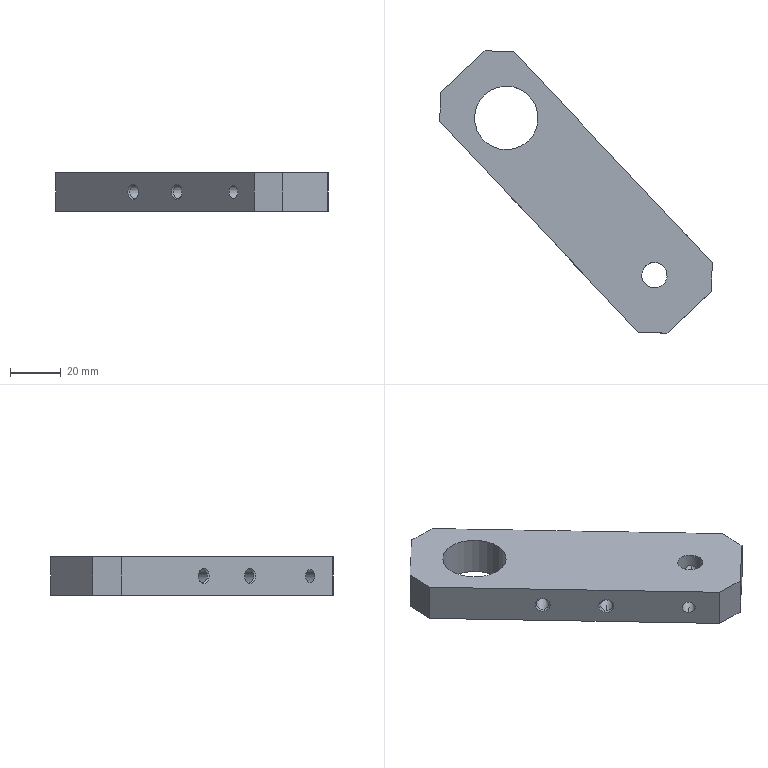Component | SolidWorks | RightSupportBlock-1 | 1 solid | 32 faces | box 107.26 x 111.11 x 15 mm | volume 66131 mm3 | cylinder 12 | cone 10 | plane 10 | commonest cylinder face diameters 5 x8 10 x2 25 x2
STEP:
#1=COLOUR_RGB('',0.7922,0.8196,0.9333);
#2=FILL_AREA_STYLE_COLOUR('',#1);
#3=FILL_AREA_STYLE('',(#2));
#4=SURFACE_STYLE_FILL_AREA(#3);
#5=SURFACE_SIDE_STYLE('',(#4));
#6=SURFACE_STYLE_USAGE(.BOTH.,#5);
#7=PRESENTATION_STYLE_ASSIGNMENT((#6));
#8=CARTESIAN_POINT('',(13.378,19.662,-9.461));
#9=VERTEX_POINT('',#8);
#10=CARTESIAN_POINT('',(13.378,19.662,-9.657));
#11=VERTEX_POINT('',#10);
#12=CARTESIAN_POINT('',(13.378,19.662,-9.559));
#13=DIRECTION('',(-0.7282,-0.6854,0.));
#14=DIRECTION('',(0.,0.,-1.));
#15=AXIS2_PLACEMENT_3D('',#12,#13,#14);
#16=CIRCLE('',#15,0.09843);
#17=EDGE_CURVE('',#9,#11,#16,.T.);
#18=ORIENTED_EDGE('',*,*,#17,.F.);
#19=CARTESIAN_POINT('',(13.363,19.648,-9.44));
#20=VERTEX_POINT('',#19);
#21=CARTESIAN_POINT('',(13.378,19.662,-9.461));
#22=DIRECTION('',(-0.5149,-0.4846,0.7071));
#23=VECTOR('',#22,39.37);
#24=LINE('',#21,#23);
#25=EDGE_CURVE('',#9,#20,#24,.T.);
#26=ORIENTED_EDGE('',*,*,#25,.T.);
#27=CARTESIAN_POINT('',(13.363,19.648,-9.678));
#28=VERTEX_POINT('',#27);
#29=CARTESIAN_POINT('',(13.363,19.648,-9.559));
#30=DIRECTION('',(0.7282,0.6854,-0.));
#31=DIRECTION('',(0.,0.,-1.));
#32=AXIS2_PLACEMENT_3D('',#29,#30,#31);
#33=CIRCLE('',#32,0.1191);
#34=EDGE_CURVE('',#28,#20,#33,.T.);
#35=ORIENTED_EDGE('',*,*,#34,.F.);
#36=CARTESIAN_POINT('',(13.378,19.662,-9.657));
#37=DIRECTION('',(-0.5149,-0.4846,-0.7071));
#38=VECTOR('',#37,39.37);
#39=LINE('',#36,#38);
#40=EDGE_CURVE('',#11,#28,#39,.T.);
#41=ORIENTED_EDGE('',*,*,#40,.F.);
#42=EDGE_LOOP('',(#18,#26,#35,#41));
#43=FACE_OUTER_BOUND('',#42,.T.);
#44=CARTESIAN_POINT('',(13.378,19.662,-9.559));
#45=DIRECTION('',(-0.7282,-0.6854,0.));
#46=DIRECTION('',(0.,0.,-1.));
#47=AXIS2_PLACEMENT_3D('',#44,#45,#46);
#48=CONICAL_SURFACE('',#47,0.09843,0.7854);
#49=ADVANCED_FACE('',(#43),#48,.F.);
#50=CARTESIAN_POINT('',(12.703,20.379,-9.461));
#51=VERTEX_POINT('',#50);
#52=CARTESIAN_POINT('',(12.703,20.379,-9.657));
#53=VERTEX_POINT('',#52);
#54=CARTESIAN_POINT('',(12.703,20.379,-9.559));
#55=DIRECTION('',(-0.7282,-0.6854,0.));
#56=DIRECTION('',(0.,0.,-1.));
#57=AXIS2_PLACEMENT_3D('',#54,#55,#56);
#58=CIRCLE('',#57,0.09843);
#59=EDGE_CURVE('',#51,#53,#58,.T.);
#60=ORIENTED_EDGE('',*,*,#59,.F.);
#61=CARTESIAN_POINT('',(12.688,20.365,-9.44));
#62=VERTEX_POINT('',#61);
#63=CARTESIAN_POINT('',(12.703,20.379,-9.461));
#64=DIRECTION('',(-0.5149,-0.4846,0.7071));
#65=VECTOR('',#64,39.37);
#66=LINE('',#63,#65);
#67=EDGE_CURVE('',#51,#62,#66,.T.);
#68=ORIENTED_EDGE('',*,*,#67,.T.);
#69=CARTESIAN_POINT('',(12.688,20.365,-9.678));
#70=VERTEX_POINT('',#69);
#71=CARTESIAN_POINT('',(12.688,20.365,-9.559));
#72=DIRECTION('',(0.7282,0.6854,-0.));
#73=DIRECTION('',(0.,0.,-1.));
#74=AXIS2_PLACEMENT_3D('',#71,#72,#73);
#75=CIRCLE('',#74,0.1191);
#76=EDGE_CURVE('',#70,#62,#75,.T.);
#77=ORIENTED_EDGE('',*,*,#76,.F.);
#78=CARTESIAN_POINT('',(12.703,20.379,-9.657));
#79=DIRECTION('',(-0.5149,-0.4846,-0.7071));
#80=VECTOR('',#79,39.37);
#81=LINE('',#78,#80);
#82=EDGE_CURVE('',#53,#70,#81,.T.);
#83=ORIENTED_EDGE('',*,*,#82,.F.);
#84=EDGE_LOOP('',(#60,#68,#77,#83));
#85=FACE_OUTER_BOUND('',#84,.T.);
#86=CARTESIAN_POINT('',(12.703,20.379,-9.559));
#87=DIRECTION('',(-0.7282,-0.6854,0.));
#88=DIRECTION('',(0.,0.,-1.));
#89=AXIS2_PLACEMENT_3D('',#86,#87,#88);
#90=CONICAL_SURFACE('',#89,0.09843,0.7854);
#91=ADVANCED_FACE('',(#85),#90,.F.);
#92=CARTESIAN_POINT('',(15.372,19.782,-9.657));
#93=VERTEX_POINT('',#92);
#94=CARTESIAN_POINT('',(15.372,19.782,-9.461));
#95=VERTEX_POINT('',#94);
#96=CARTESIAN_POINT('',(15.372,19.782,-9.559));
#97=DIRECTION('',(0.7282,0.6854,-0.));
#98=DIRECTION('',(0.,0.,1.));
#99=AXIS2_PLACEMENT_3D('',#96,#97,#98);
#100=CIRCLE('',#99,0.09843);
#101=EDGE_CURVE('',#93,#95,#100,.T.);
#102=ORIENTED_EDGE('',*,*,#101,.F.);
#103=CARTESIAN_POINT('',(15.387,19.796,-9.678));
#104=VERTEX_POINT('',#103);
#105=CARTESIAN_POINT('',(15.372,19.782,-9.657));
#106=DIRECTION('',(0.5149,0.4846,-0.7071));
#107=VECTOR('',#106,39.37);
#108=LINE('',#105,#107);
#109=EDGE_CURVE('',#93,#104,#108,.T.);
#110=ORIENTED_EDGE('',*,*,#109,.T.);
#111=CARTESIAN_POINT('',(15.387,19.796,-9.44));
#112=VERTEX_POINT('',#111);
#113=CARTESIAN_POINT('',(15.387,19.796,-9.559));
#114=DIRECTION('',(-0.7282,-0.6854,0.));
#115=DIRECTION('',(-0.6854,0.7282,0.));
#116=AXIS2_PLACEMENT_3D('',#113,#114,#115);
#117=CIRCLE('',#116,0.1191);
#118=EDGE_CURVE('',#112,#104,#117,.T.);
#119=ORIENTED_EDGE('',*,*,#118,.F.);
#120=CARTESIAN_POINT('',(15.372,19.782,-9.461));
#121=DIRECTION('',(0.5149,0.4846,0.7071));
#122=VECTOR('',#121,39.37);
#123=LINE('',#120,#122);
#124=EDGE_CURVE('',#95,#112,#123,.T.);
#125=ORIENTED_EDGE('',*,*,#124,.F.);
#126=EDGE_LOOP('',(#102,#110,#119,#125));
#127=FACE_OUTER_BOUND('',#126,.T.);
#128=CARTESIAN_POINT('',(15.372,19.782,-9.559));
#129=DIRECTION('',(0.7282,0.6854,-0.));
#130=DIRECTION('',(0.,0.,1.));
#131=AXIS2_PLACEMENT_3D('',#128,#129,#130);
#132=CONICAL_SURFACE('',#131,0.09843,0.7854);
#133=ADVANCED_FACE('',(#127),#132,.F.);
#134=CARTESIAN_POINT('',(13.262,20.905,-9.461));
#135=VERTEX_POINT('',#134);
#136=CARTESIAN_POINT('',(13.262,20.905,-9.657));
#137=VERTEX_POINT('',#136);
#138=CARTESIAN_POINT('',(13.262,20.905,-9.559));
#139=DIRECTION('',(-0.7282,-0.6854,0.));
#140=DIRECTION('',(0.,0.,-1.));
#141=AXIS2_PLACEMENT_3D('',#138,#139,#140);
#142=CIRCLE('',#141,0.09843);
#143=EDGE_CURVE('',#135,#137,#142,.T.);
#144=ORIENTED_EDGE('',*,*,#143,.F.);
#145=CARTESIAN_POINT('',(12.688,20.365,-9.461));
#146=DIRECTION('',(-0.7282,-0.6854,0.));
#147=VECTOR('',#146,39.37);
#148=LINE('',#145,#147);
#149=EDGE_CURVE('',#135,#51,#148,.T.);
#150=ORIENTED_EDGE('',*,*,#149,.T.);
#151=ORIENTED_EDGE('',*,*,#59,.T.);
#152=CARTESIAN_POINT('',(12.688,20.365,-9.657));
#153=DIRECTION('',(-0.7282,-0.6854,0.));
#154=VECTOR('',#153,39.37);
#155=LINE('',#152,#154);
#156=EDGE_CURVE('',#137,#53,#155,.T.);
#157=ORIENTED_EDGE('',*,*,#156,.F.);
#158=EDGE_LOOP('',(#144,#150,#151,#157));
#159=FACE_OUTER_BOUND('',#158,.T.);
#160=CARTESIAN_POINT('',(12.688,20.365,-9.559));
#161=DIRECTION('',(-0.7282,-0.6854,0.));
#162=DIRECTION('',(0.,0.,-1.));
#163=AXIS2_PLACEMENT_3D('',#160,#161,#162);
#164=CYLINDRICAL_SURFACE('',#163,0.09843);
#165=ADVANCED_FACE('',(#159),#164,.F.);
#166=CARTESIAN_POINT('',(13.305,20.945,-9.559));
#167=VERTEX_POINT('',#166);
#168=CARTESIAN_POINT('',(13.262,20.905,-9.657));
#169=DIRECTION('',(-0.375,-0.353,-0.8572));
#170=VECTOR('',#169,39.37);
#171=LINE('',#168,#170);
#172=EDGE_CURVE('',#167,#137,#171,.T.);
#173=ORIENTED_EDGE('',*,*,#172,.F.);
#174=CARTESIAN_POINT('',(13.262,20.905,-9.461));
#175=DIRECTION('',(-0.375,-0.353,0.8572));
#176=VECTOR('',#175,39.37);
#177=LINE('',#174,#176);
#178=EDGE_CURVE('',#167,#135,#177,.T.);
#179=ORIENTED_EDGE('',*,*,#178,.T.);
#180=ORIENTED_EDGE('',*,*,#143,.T.);
#181=EDGE_LOOP('',(#173,#179,#180));
#182=FACE_OUTER_BOUND('',#181,.T.);
#183=CARTESIAN_POINT('',(13.262,20.905,-9.559));
#184=DIRECTION('',(-0.7282,-0.6854,0.));
#185=DIRECTION('',(0.,0.,-1.));
#186=AXIS2_PLACEMENT_3D('',#183,#184,#185);
#187=CONICAL_SURFACE('',#186,0.09843,1.03);
#188=ADVANCED_FACE('',(#182),#187,.F.);
#189=CARTESIAN_POINT('',(13.936,20.188,-9.461));
#190=VERTEX_POINT('',#189);
#191=CARTESIAN_POINT('',(13.936,20.188,-9.657));
#192=VERTEX_POINT('',#191);
#193=CARTESIAN_POINT('',(13.936,20.188,-9.559));
#194=DIRECTION('',(-0.7282,-0.6854,0.));
#195=DIRECTION('',(0.,0.,-1.));
#196=AXIS2_PLACEMENT_3D('',#193,#194,#195);
#197=CIRCLE('',#196,0.09843);
#198=EDGE_CURVE('',#190,#192,#197,.T.);
#199=ORIENTED_EDGE('',*,*,#198,.F.);
#200=CARTESIAN_POINT('',(13.363,19.648,-9.461));
#201=DIRECTION('',(-0.7282,-0.6854,0.));
#202=VECTOR('',#201,39.37);
#203=LINE('',#200,#202);
#204=EDGE_CURVE('',#190,#9,#203,.T.);
#205=ORIENTED_EDGE('',*,*,#204,.T.);
#206=ORIENTED_EDGE('',*,*,#17,.T.);
#207=CARTESIAN_POINT('',(13.363,19.648,-9.657));
#208=DIRECTION('',(-0.7282,-0.6854,0.));
#209=VECTOR('',#208,39.37);
#210=LINE('',#207,#209);
#211=EDGE_CURVE('',#192,#11,#210,.T.);
#212=ORIENTED_EDGE('',*,*,#211,.F.);
#213=EDGE_LOOP('',(#199,#205,#206,#212));
#214=FACE_OUTER_BOUND('',#213,.T.);
#215=CARTESIAN_POINT('',(13.363,19.648,-9.559));
#216=DIRECTION('',(-0.7282,-0.6854,0.));
#217=DIRECTION('',(0.,0.,-1.));
#218=AXIS2_PLACEMENT_3D('',#215,#216,#217);
#219=CYLINDRICAL_SURFACE('',#218,0.09843);
#220=ADVANCED_FACE('',(#214),#219,.F.);
#221=CARTESIAN_POINT('',(13.979,20.228,-9.559));
#222=VERTEX_POINT('',#221);
#223=CARTESIAN_POINT('',(13.936,20.188,-9.657));
#224=DIRECTION('',(-0.375,-0.353,-0.8572));
#225=VECTOR('',#224,39.37);
#226=LINE('',#223,#225);
#227=EDGE_CURVE('',#222,#192,#226,.T.);
#228=ORIENTED_EDGE('',*,*,#227,.F.);
#229=CARTESIAN_POINT('',(13.936,20.188,-9.461));
#230=DIRECTION('',(-0.375,-0.353,0.8572));
#231=VECTOR('',#230,39.37);
#232=LINE('',#229,#231);
#233=EDGE_CURVE('',#222,#190,#232,.T.);
#234=ORIENTED_EDGE('',*,*,#233,.T.);
#235=ORIENTED_EDGE('',*,*,#198,.T.);
#236=EDGE_LOOP('',(#228,#234,#235));
#237=FACE_OUTER_BOUND('',#236,.T.);
#238=CARTESIAN_POINT('',(13.936,20.188,-9.559));
#239=DIRECTION('',(-0.7282,-0.6854,0.));
#240=DIRECTION('',(0.,0.,-1.));
#241=AXIS2_PLACEMENT_3D('',#238,#239,#240);
#242=CONICAL_SURFACE('',#241,0.09843,1.03);
#243=ADVANCED_FACE('',(#237),#242,.F.);
#244=CARTESIAN_POINT('',(14.24,18.716,-9.461));
#245=VERTEX_POINT('',#244);
#246=CARTESIAN_POINT('',(14.24,18.716,-9.657));
#247=VERTEX_POINT('',#246);
#248=CARTESIAN_POINT('',(14.24,18.716,-9.559));
#249=DIRECTION('',(-0.7282,-0.6854,0.));
#250=DIRECTION('',(0.,0.,-1.));
#251=AXIS2_PLACEMENT_3D('',#248,#249,#250);
#252=CIRCLE('',#251,0.09843);
#253=EDGE_CURVE('',#245,#247,#252,.T.);
#254=ORIENTED_EDGE('',*,*,#253,.T.);
#255=CARTESIAN_POINT('',(14.67,19.121,-9.657));
#256=VERTEX_POINT('',#255);
#257=CARTESIAN_POINT('',(15.387,19.796,-9.657));
#258=DIRECTION('',(0.7282,0.6854,-0.));
#259=VECTOR('',#258,39.37);
#260=LINE('',#257,#259);
#261=EDGE_CURVE('',#247,#256,#260,.T.);
#262=ORIENTED_EDGE('',*,*,#261,.T.);
#263=CARTESIAN_POINT('',(14.67,19.121,-9.461));
#264=VERTEX_POINT('',#263);
#265=CARTESIAN_POINT('',(14.67,19.121,-9.461));
#266=CARTESIAN_POINT('',(14.665,19.126,-9.461));
#267=CARTESIAN_POINT('',(14.661,19.131,-9.461));
#268=CARTESIAN_POINT('',(14.653,19.141,-9.464));
#269=CARTESIAN_POINT('',(14.65,19.146,-9.466));
#270=CARTESIAN_POINT('',(14.64,19.162,-9.473));
#271=CARTESIAN_POINT('',(14.635,19.172,-9.481));
#272=CARTESIAN_POINT('',(14.63,19.185,-9.494));
#273=CARTESIAN_POINT('',(14.628,19.189,-9.499));
#274=CARTESIAN_POINT('',(14.626,19.197,-9.51));
#275=CARTESIAN_POINT('',(14.625,19.2,-9.515));
#276=CARTESIAN_POINT('',(14.623,19.205,-9.527));
#277=CARTESIAN_POINT('',(14.623,19.207,-9.533));
#278=CARTESIAN_POINT('',(14.622,19.21,-9.546));
#279=CARTESIAN_POINT('',(14.622,19.211,-9.552));
#280=CARTESIAN_POINT('',(14.622,19.211,-9.566));
#281=CARTESIAN_POINT('',(14.622,19.21,-9.572));
#282=CARTESIAN_POINT('',(14.623,19.207,-9.585));
#283=CARTESIAN_POINT('',(14.623,19.205,-9.591));
#284=CARTESIAN_POINT('',(14.625,19.2,-9.603));
#285=CARTESIAN_POINT('',(14.626,19.197,-9.609));
#286=CARTESIAN_POINT('',(14.628,19.189,-9.619));
#287=CARTESIAN_POINT('',(14.63,19.185,-9.624));
#288=CARTESIAN_POINT('',(14.635,19.172,-9.638));
#289=CARTESIAN_POINT('',(14.64,19.162,-9.645));
#290=CARTESIAN_POINT('',(14.65,19.146,-9.652));
#291=CARTESIAN_POINT('',(14.653,19.141,-9.654));
#292=CARTESIAN_POINT('',(14.661,19.131,-9.657));
#293=CARTESIAN_POINT('',(14.665,19.126,-9.657));
#294=CARTESIAN_POINT('',(14.67,19.121,-9.657));
#295=B_SPLINE_CURVE_WITH_KNOTS('',3,(#265,#266,#267,#268,#269,#270,#271,#272,#273,#274,#275,#276,#277,#278,#279,#280,#281,#282,#283,#284,#285,#286,#287,#288,#289,#290,#291,#292,#293,#294),.UNSPECIFIED.,.F.,.F.,(4,2,2,2,2,2,2,2,2,2,2,2,2,2,4),(0.,0.000497,0.0009941,0.001988,0.002485,0.002982,0.003479,0.003976,0.004473,0.00497,0.005467,0.005964,0.006958,0.007455,0.007952),.UNSPECIFIED.);
#296=EDGE_CURVE('',#264,#256,#295,.T.);
#297=ORIENTED_EDGE('',*,*,#296,.F.);
#298=CARTESIAN_POINT('',(15.387,19.796,-9.461));
#299=DIRECTION('',(0.7282,0.6854,-0.));
#300=VECTOR('',#299,39.37);
#301=LINE('',#298,#300);
#302=EDGE_CURVE('',#245,#264,#301,.T.);
#303=ORIENTED_EDGE('',*,*,#302,.F.);
#304=EDGE_LOOP('',(#254,#262,#297,#303));
#305=FACE_OUTER_BOUND('',#304,.T.);
#306=CARTESIAN_POINT('',(15.387,19.796,-9.559));
#307=DIRECTION('',(0.7282,0.6854,-0.));
#308=DIRECTION('',(0.,0.,1.));
#309=AXIS2_PLACEMENT_3D('',#306,#307,#308);
#310=CYLINDRICAL_SURFACE('',#309,0.09843);
#311=ADVANCED_FACE('',(#305),#310,.F.);
#312=CARTESIAN_POINT('',(14.957,19.391,-9.657));
#313=VERTEX_POINT('',#312);
#314=CARTESIAN_POINT('',(14.957,19.391,-9.461));
#315=VERTEX_POINT('',#314);
#316=CARTESIAN_POINT('',(14.957,19.391,-9.657));
#317=CARTESIAN_POINT('',(14.952,19.396,-9.657));
#318=CARTESIAN_POINT('',(14.947,19.4,-9.657));
#319=CARTESIAN_POINT('',(14.938,19.409,-9.654));
#320=CARTESIAN_POINT('',(14.933,19.413,-9.652));
#321=CARTESIAN_POINT('',(14.923,19.42,-9.647));
#322=CARTESIAN_POINT('',(14.918,19.423,-9.644));
#323=CARTESIAN_POINT('',(14.909,19.428,-9.637));
#324=CARTESIAN_POINT('',(14.904,19.431,-9.633));
#325=CARTESIAN_POINT('',(14.895,19.435,-9.624));
#326=CARTESIAN_POINT('',(14.891,19.437,-9.619));
#327=CARTESIAN_POINT('',(14.884,19.44,-9.609));
#328=CARTESIAN_POINT('',(14.881,19.441,-9.603));
#329=CARTESIAN_POINT('',(14.876,19.443,-9.591));
#330=CARTESIAN_POINT('',(14.874,19.443,-9.585));
#331=CARTESIAN_POINT('',(14.871,19.444,-9.572));
#332=CARTESIAN_POINT('',(14.87,19.445,-9.566));
#333=CARTESIAN_POINT('',(14.87,19.445,-9.553));
#334=CARTESIAN_POINT('',(14.871,19.444,-9.546));
#335=CARTESIAN_POINT('',(14.874,19.444,-9.533));
#336=CARTESIAN_POINT('',(14.876,19.443,-9.527));
#337=CARTESIAN_POINT('',(14.884,19.44,-9.509));
#338=CARTESIAN_POINT('',(14.891,19.437,-9.499));
#339=CARTESIAN_POINT('',(14.904,19.431,-9.485));
#340=CARTESIAN_POINT('',(14.908,19.428,-9.481));
#341=CARTESIAN_POINT('',(14.918,19.423,-9.474));
#342=CARTESIAN_POINT('',(14.923,19.42,-9.471));
#343=CARTESIAN_POINT('',(14.933,19.413,-9.466));
#344=CARTESIAN_POINT('',(14.938,19.409,-9.464));
#345=CARTESIAN_POINT('',(14.947,19.4,-9.461));
#346=CARTESIAN_POINT('',(14.952,19.396,-9.461));
#347=CARTESIAN_POINT('',(14.957,19.391,-9.461));
#348=B_SPLINE_CURVE_WITH_KNOTS('',3,(#316,#317,#318,#319,#320,#321,#322,#323,#324,#325,#326,#327,#328,#329,#330,#331,#332,#333,#334,#335,#336,#337,#338,#339,#340,#341,#342,#343,#344,#345,#346,#347),.UNSPECIFIED.,.F.,.F.,(4,2,2,2,2,2,2,2,2,2,2,2,2,2,2,4),(0.007952,0.008449,0.008945,0.009441,0.009937,0.01043,0.01093,0.01143,0.01192,0.01242,0.01291,0.01391,0.0144,0.0149,0.01539,0.01589),.UNSPECIFIED.);
#349=EDGE_CURVE('',#313,#315,#348,.T.);
#350=ORIENTED_EDGE('',*,*,#349,.F.);
#351=CARTESIAN_POINT('',(15.387,19.796,-9.657));
#352=DIRECTION('',(0.7282,0.6854,-0.));
#353=VECTOR('',#352,39.37);
#354=LINE('',#351,#353);
#355=EDGE_CURVE('',#313,#93,#354,.T.);
#356=ORIENTED_EDGE('',*,*,#355,.T.);
#357=ORIENTED_EDGE('',*,*,#101,.T.);
#358=CARTESIAN_POINT('',(15.387,19.796,-9.461));
#359=DIRECTION('',(0.7282,0.6854,-0.));
#360=VECTOR('',#359,39.37);
#361=LINE('',#358,#360);
#362=EDGE_CURVE('',#315,#95,#361,.T.);
#363=ORIENTED_EDGE('',*,*,#362,.F.);
#364=EDGE_LOOP('',(#350,#356,#357,#363));
#365=FACE_OUTER_BOUND('',#364,.T.);
#366=CARTESIAN_POINT('',(15.387,19.796,-9.559));
#367=DIRECTION('',(0.7282,0.6854,-0.));
#368=DIRECTION('',(0.,0.,1.));
#369=AXIS2_PLACEMENT_3D('',#366,#367,#368);
#370=CYLINDRICAL_SURFACE('',#369,0.09843);
#371=ADVANCED_FACE('',(#365),#370,.F.);
#372=ORIENTED_EDGE('',*,*,#296,.T.);
#373=CARTESIAN_POINT('',(14.67,19.121,-9.657));
#374=CARTESIAN_POINT('',(14.674,19.116,-9.657));
#375=CARTESIAN_POINT('',(14.679,19.112,-9.657));
#376=CARTESIAN_POINT('',(14.689,19.103,-9.654));
#377=CARTESIAN_POINT('',(14.694,19.1,-9.652));
#378=CARTESIAN_POINT('',(14.704,19.092,-9.647));
#379=CARTESIAN_POINT('',(14.709,19.089,-9.644));
#380=CARTESIAN_POINT('',(14.718,19.084,-9.637));
#381=CARTESIAN_POINT('',(14.723,19.081,-9.633));
#382=CARTESIAN_POINT('',(14.731,19.077,-9.624));
#383=CARTESIAN_POINT('',(14.735,19.075,-9.619));
#384=CARTESIAN_POINT('',(14.742,19.072,-9.609));
#385=CARTESIAN_POINT('',(14.746,19.071,-9.603));
#386=CARTESIAN_POINT('',(14.751,19.069,-9.591));
#387=CARTESIAN_POINT('',(14.753,19.069,-9.585));
#388=CARTESIAN_POINT('',(14.756,19.068,-9.572));
#389=CARTESIAN_POINT('',(14.757,19.068,-9.566));
#390=CARTESIAN_POINT('',(14.757,19.068,-9.553));
#391=CARTESIAN_POINT('',(14.756,19.068,-9.546));
#392=CARTESIAN_POINT('',(14.753,19.069,-9.533));
#393=CARTESIAN_POINT('',(14.751,19.069,-9.527));
#394=CARTESIAN_POINT('',(14.743,19.072,-9.509));
#395=CARTESIAN_POINT('',(14.736,19.075,-9.499));
#396=CARTESIAN_POINT('',(14.723,19.081,-9.485));
#397=CARTESIAN_POINT('',(14.718,19.084,-9.481));
#398=CARTESIAN_POINT('',(14.709,19.089,-9.474));
#399=CARTESIAN_POINT('',(14.704,19.092,-9.471));
#400=CARTESIAN_POINT('',(14.694,19.099,-9.466));
#401=CARTESIAN_POINT('',(14.689,19.103,-9.464));
#402=CARTESIAN_POINT('',(14.679,19.112,-9.461));
#403=CARTESIAN_POINT('',(14.674,19.116,-9.461));
#404=CARTESIAN_POINT('',(14.67,19.121,-9.461));
#405=B_SPLINE_CURVE_WITH_KNOTS('',3,(#373,#374,#375,#376,#377,#378,#379,#380,#381,#382,#383,#384,#385,#386,#387,#388,#389,#390,#391,#392,#393,#394,#395,#396,#397,#398,#399,#400,#401,#402,#403,#404),.UNSPECIFIED.,.F.,.F.,(4,2,2,2,2,2,2,2,2,2,2,2,2,2,2,4),(0.007952,0.008449,0.008945,0.009441,0.009937,0.01043,0.01093,0.01143,0.01192,0.01242,0.01291,0.01391,0.0144,0.0149,0.01539,0.01589),.UNSPECIFIED.);
#406=EDGE_CURVE('',#256,#264,#405,.T.);
#407=ORIENTED_EDGE('',*,*,#406,.T.);
#408=EDGE_LOOP('',(#372,#407));
#409=FACE_BOUND('',#408,.T.);
#410=CARTESIAN_POINT('',(14.678,19.399,-9.854));
#411=VERTEX_POINT('',#410);
#412=CARTESIAN_POINT('',(14.948,19.113,-9.854));
#413=VERTEX_POINT('',#412);
#414=CARTESIAN_POINT('',(14.813,19.256,-9.854));
#415=DIRECTION('',(-0.,0.,1.));
#416=DIRECTION('',(0.6854,-0.7282,0.));
#417=AXIS2_PLACEMENT_3D('',#414,#415,#416);
#418=CIRCLE('',#417,0.1969);
#419=EDGE_CURVE('',#411,#413,#418,.T.);
#420=ORIENTED_EDGE('',*,*,#419,.F.);
#421=CARTESIAN_POINT('',(14.678,19.399,-9.264));
#422=VERTEX_POINT('',#421);
#423=CARTESIAN_POINT('',(14.678,19.399,-9.264));
#424=DIRECTION('',(-0.,0.,1.));
#425=VECTOR('',#424,39.37);
#426=LINE('',#423,#425);
#427=EDGE_CURVE('',#411,#422,#426,.T.);
#428=ORIENTED_EDGE('',*,*,#427,.T.);
#429=CARTESIAN_POINT('',(14.948,19.113,-9.264));
#430=VERTEX_POINT('',#429);
#431=CARTESIAN_POINT('',(14.813,19.256,-9.264));
#432=DIRECTION('',(-0.,0.,1.));
#433=DIRECTION('',(0.6854,-0.7282,0.));
#434=AXIS2_PLACEMENT_3D('',#431,#432,#433);
#435=CIRCLE('',#434,0.1969);
#436=EDGE_CURVE('',#422,#430,#435,.T.);
#437=ORIENTED_EDGE('',*,*,#436,.T.);
#438=CARTESIAN_POINT('',(14.948,19.113,-9.264));
#439=DIRECTION('',(-0.,0.,1.));
#440=VECTOR('',#439,39.37);
#441=LINE('',#438,#440);
#442=EDGE_CURVE('',#413,#430,#441,.T.);
#443=ORIENTED_EDGE('',*,*,#442,.F.);
#444=EDGE_LOOP('',(#420,#428,#437,#443));
#445=FACE_OUTER_BOUND('',#444,.T.);
#446=CARTESIAN_POINT('',(14.813,19.256,-9.264));
#447=DIRECTION('',(-0.,0.,1.));
#448=DIRECTION('',(0.6854,-0.7282,0.));
#449=AXIS2_PLACEMENT_3D('',#446,#447,#448);
#450=CYLINDRICAL_SURFACE('',#449,0.1969);
#451=ADVANCED_FACE('',(#409,#445),#450,.F.);
#452=CARTESIAN_POINT('',(12.182,22.051,-9.854));
#453=VERTEX_POINT('',#452);
#454=CARTESIAN_POINT('',(12.857,21.335,-9.854));
#455=VERTEX_POINT('',#454);
#456=CARTESIAN_POINT('',(12.52,21.693,-9.854));
#457=DIRECTION('',(-0.,0.,1.));
#458=DIRECTION('',(0.6854,-0.7282,0.));
#459=AXIS2_PLACEMENT_3D('',#456,#457,#458);
#460=CIRCLE('',#459,0.4921);
#461=EDGE_CURVE('',#453,#455,#460,.T.);
#462=ORIENTED_EDGE('',*,*,#461,.F.);
#463=CARTESIAN_POINT('',(12.182,22.051,-9.264));
#464=VERTEX_POINT('',#463);
#465=CARTESIAN_POINT('',(12.182,22.051,-9.264));
#466=DIRECTION('',(-0.,0.,1.));
#467=VECTOR('',#466,39.37);
#468=LINE('',#465,#467);
#469=EDGE_CURVE('',#453,#464,#468,.T.);
#470=ORIENTED_EDGE('',*,*,#469,.T.);
#471=CARTESIAN_POINT('',(12.857,21.335,-9.264));
#472=VERTEX_POINT('',#471);
#473=CARTESIAN_POINT('',(12.52,21.693,-9.264));
#474=DIRECTION('',(-0.,0.,1.));
#475=DIRECTION('',(0.6854,-0.7282,0.));
#476=AXIS2_PLACEMENT_3D('',#473,#474,#475);
#477=CIRCLE('',#476,0.4921);
#478=EDGE_CURVE('',#464,#472,#477,.T.);
#479=ORIENTED_EDGE('',*,*,#478,.T.);
#480=CARTESIAN_POINT('',(12.857,21.335,-9.264));
#481=DIRECTION('',(-0.,0.,1.));
#482=VECTOR('',#481,39.37);
#483=LINE('',#480,#482);
#484=EDGE_CURVE('',#455,#472,#483,.T.);
#485=ORIENTED_EDGE('',*,*,#484,.F.);
#486=EDGE_LOOP('',(#462,#470,#479,#485));
#487=FACE_OUTER_BOUND('',#486,.T.);
#488=CARTESIAN_POINT('',(12.52,21.693,-9.264));
#489=DIRECTION('',(-0.,0.,1.));
#490=DIRECTION('',(0.6854,-0.7282,0.));
#491=AXIS2_PLACEMENT_3D('',#488,#489,#490);
#492=CYLINDRICAL_SURFACE('',#491,0.4921);
#493=ADVANCED_FACE('',(#487),#492,.F.);
#494=CARTESIAN_POINT('',(15.697,19.007,-9.264));
#495=VERTEX_POINT('',#494);
#496=CARTESIAN_POINT('',(15.009,18.359,-9.264));
#497=VERTEX_POINT('',#496);
#498=CARTESIAN_POINT('',(15.926,19.222,-9.264));
#499=DIRECTION('',(-0.7282,-0.6854,0.));
#500=VECTOR('',#499,39.37);
#501=LINE('',#498,#500);
#502=EDGE_CURVE('',#495,#497,#501,.T.);
#503=ORIENTED_EDGE('',*,*,#502,.T.);
#504=CARTESIAN_POINT('',(15.009,18.359,-9.854));
#505=VERTEX_POINT('',#504);
#506=CARTESIAN_POINT('',(15.009,18.359,-9.264));
#507=DIRECTION('',(0.,-0.,-1.));
#508=VECTOR('',#507,39.37);
#509=LINE('',#506,#508);
#510=EDGE_CURVE('',#497,#505,#509,.T.);
#511=ORIENTED_EDGE('',*,*,#510,.T.);
#512=CARTESIAN_POINT('',(15.697,19.007,-9.854));
#513=VERTEX_POINT('',#512);
#514=CARTESIAN_POINT('',(15.926,19.222,-9.854));
#515=DIRECTION('',(-0.7282,-0.6854,0.));
#516=VECTOR('',#515,39.37);
#517=LINE('',#514,#516);
#518=EDGE_CURVE('',#513,#505,#517,.T.);
#519=ORIENTED_EDGE('',*,*,#518,.F.);
#520=CARTESIAN_POINT('',(15.697,19.007,-9.264));
#521=DIRECTION('',(-0.,0.,1.));
#522=VECTOR('',#521,39.37);
#523=LINE('',#520,#522);
#524=EDGE_CURVE('',#513,#495,#523,.T.);
#525=ORIENTED_EDGE('',*,*,#524,.T.);
#526=EDGE_LOOP('',(#503,#511,#519,#525));
#527=FACE_OUTER_BOUND('',#526,.T.);
#528=CARTESIAN_POINT('',(15.926,19.222,-9.264));
#529=DIRECTION('',(0.6854,-0.7282,0.));
#530=DIRECTION('',(0.,-0.,-1.));
#531=AXIS2_PLACEMENT_3D('',#528,#529,#530);
#532=PLANE('',#531);
#533=ADVANCED_FACE('',(#527),#532,.T.);
#534=ORIENTED_EDGE('',*,*,#118,.T.);
#535=CARTESIAN_POINT('',(15.387,19.796,-9.559));
#536=DIRECTION('',(-0.7282,-0.6854,0.));
#537=DIRECTION('',(-0.6854,0.7282,0.));
#538=AXIS2_PLACEMENT_3D('',#535,#536,#537);
#539=CIRCLE('',#538,0.1191);
#540=EDGE_CURVE('',#104,#112,#539,.T.);
#541=ORIENTED_EDGE('',*,*,#540,.T.);
#542=EDGE_LOOP('',(#534,#541));
#543=FACE_BOUND('',#542,.T.);
#544=CARTESIAN_POINT('',(12.634,22.72,-9.854));
#545=VERTEX_POINT('',#544);
#546=CARTESIAN_POINT('',(15.71,19.452,-9.854));
#547=VERTEX_POINT('',#546);
#548=CARTESIAN_POINT('',(12.418,22.949,-9.854));
#549=DIRECTION('',(0.6854,-0.7282,0.));
#550=VECTOR('',#549,39.37);
#551=LINE('',#548,#550);
#552=EDGE_CURVE('',#545,#547,#551,.T.);
#553=ORIENTED_EDGE('',*,*,#552,.F.);
#554=CARTESIAN_POINT('',(12.634,22.72,-9.264));
#555=VERTEX_POINT('',#554);
#556=CARTESIAN_POINT('',(12.634,22.72,-9.264));
#557=DIRECTION('',(-0.,0.,1.));
#558=VECTOR('',#557,39.37);
#559=LINE('',#556,#558);
#560=EDGE_CURVE('',#545,#555,#559,.T.);
#561=ORIENTED_EDGE('',*,*,#560,.T.);
#562=CARTESIAN_POINT('',(15.71,19.452,-9.264));
#563=VERTEX_POINT('',#562);
#564=CARTESIAN_POINT('',(12.418,22.949,-9.264));
#565=DIRECTION('',(0.6854,-0.7282,0.));
#566=VECTOR('',#565,39.37);
#567=LINE('',#564,#566);
#568=EDGE_CURVE('',#555,#563,#567,.T.);
#569=ORIENTED_EDGE('',*,*,#568,.T.);
#570=CARTESIAN_POINT('',(15.71,19.452,-9.264));
#571=DIRECTION('',(0.,-0.,-1.));
#572=VECTOR('',#571,39.37);
#573=LINE('',#570,#572);
#574=EDGE_CURVE('',#563,#547,#573,.T.);
#575=ORIENTED_EDGE('',*,*,#574,.T.);
#576=EDGE_LOOP('',(#553,#561,#569,#575));
#577=FACE_OUTER_BOUND('',#576,.T.);
#578=CARTESIAN_POINT('',(12.418,22.949,-9.264));
#579=DIRECTION('',(0.7282,0.6854,-0.));
#580=DIRECTION('',(-0.6854,0.7282,-0.));
#581=AXIS2_PLACEMENT_3D('',#578,#579,#580);
#582=PLANE('',#581);
#583=ADVANCED_FACE('',(#543,#577),#582,.T.);
#584=CARTESIAN_POINT('',(11.501,22.086,-9.854));
#585=VERTEX_POINT('',#584);
#586=CARTESIAN_POINT('',(12.189,22.733,-9.854));
#587=VERTEX_POINT('',#586);
#588=CARTESIAN_POINT('',(11.272,21.87,-9.854));
#589=DIRECTION('',(0.7282,0.6854,-0.));
#590=VECTOR('',#589,39.37);
#591=LINE('',#588,#590);
#592=EDGE_CURVE('',#585,#587,#591,.T.);
#593=ORIENTED_EDGE('',*,*,#592,.F.);
#594=CARTESIAN_POINT('',(11.501,22.086,-9.264));
#595=VERTEX_POINT('',#594);
#596=CARTESIAN_POINT('',(11.501,22.086,-9.264));
#597=DIRECTION('',(-0.,0.,1.));
#598=VECTOR('',#597,39.37);
#599=LINE('',#596,#598);
#600=EDGE_CURVE('',#585,#595,#599,.T.);
#601=ORIENTED_EDGE('',*,*,#600,.T.);
#602=CARTESIAN_POINT('',(12.189,22.733,-9.264));
#603=VERTEX_POINT('',#602);
#604=CARTESIAN_POINT('',(11.272,21.87,-9.264));
#605=DIRECTION('',(0.7282,0.6854,-0.));
#606=VECTOR('',#605,39.37);
#607=LINE('',#604,#606);
#608=EDGE_CURVE('',#595,#603,#607,.T.);
#609=ORIENTED_EDGE('',*,*,#608,.T.);
#610=CARTESIAN_POINT('',(12.189,22.733,-9.264));
#611=DIRECTION('',(0.,-0.,-1.));
#612=VECTOR('',#611,39.37);
#613=LINE('',#610,#612);
#614=EDGE_CURVE('',#603,#587,#613,.T.);
#615=ORIENTED_EDGE('',*,*,#614,.T.);
#616=EDGE_LOOP('',(#593,#601,#609,#615));
#617=FACE_OUTER_BOUND('',#616,.T.);
#618=CARTESIAN_POINT('',(11.272,21.87,-9.264));
#619=DIRECTION('',(-0.6854,0.7282,-0.));
#620=DIRECTION('',(-0.,0.,1.));
#621=AXIS2_PLACEMENT_3D('',#618,#619,#620);
#622=PLANE('',#621);
#623=ADVANCED_FACE('',(#617),#622,.T.);
#624=ORIENTED_EDGE('',*,*,#76,.T.);
#625=CARTESIAN_POINT('',(12.688,20.365,-9.559));
#626=DIRECTION('',(0.7282,0.6854,-0.));
#627=DIRECTION('',(-0.,0.,-1.));
#628=AXIS2_PLACEMENT_3D('',#625,#626,#627);
#629=CIRCLE('',#628,0.1191);
#630=EDGE_CURVE('',#62,#70,#629,.T.);
#631=ORIENTED_EDGE('',*,*,#630,.T.);
#632=EDGE_LOOP('',(#624,#631));
#633=FACE_BOUND('',#632,.T.);
#634=ORIENTED_EDGE('',*,*,#34,.T.);
#635=CARTESIAN_POINT('',(13.363,19.648,-9.559));
#636=DIRECTION('',(0.7282,0.6854,-0.));
#637=DIRECTION('',(0.,0.,-1.));
#638=AXIS2_PLACEMENT_3D('',#635,#636,#637);
#639=CIRCLE('',#638,0.1191);
#640=EDGE_CURVE('',#20,#28,#639,.T.);
#641=ORIENTED_EDGE('',*,*,#640,.T.);
#642=EDGE_LOOP('',(#634,#641));
#643=FACE_BOUND('',#642,.T.);
#644=ORIENTED_EDGE('',*,*,#253,.F.);
#645=CARTESIAN_POINT('',(14.24,18.716,-9.559));
#646=DIRECTION('',(-0.7282,-0.6854,0.));
#647=DIRECTION('',(0.,0.,-1.));
#648=AXIS2_PLACEMENT_3D('',#645,#646,#647);
#649=CIRCLE('',#648,0.09843);
#650=EDGE_CURVE('',#247,#245,#649,.T.);
#651=ORIENTED_EDGE('',*,*,#650,.F.);
#652=EDGE_LOOP('',(#644,#651));
#653=FACE_BOUND('',#652,.T.);
#654=CARTESIAN_POINT('',(14.564,18.372,-9.264));
#655=VERTEX_POINT('',#654);
#656=CARTESIAN_POINT('',(11.488,21.641,-9.264));
#657=VERTEX_POINT('',#656);
#658=CARTESIAN_POINT('',(14.78,18.143,-9.264));
#659=DIRECTION('',(-0.6854,0.7282,-0.));
#660=VECTOR('',#659,39.37);
#661=LINE('',#658,#660);
#662=EDGE_CURVE('',#655,#657,#661,.T.);
#663=ORIENTED_EDGE('',*,*,#662,.T.);
#664=CARTESIAN_POINT('',(11.488,21.641,-9.854));
#665=VERTEX_POINT('',#664);
#666=CARTESIAN_POINT('',(11.488,21.641,-9.264));
#667=DIRECTION('',(0.,-0.,-1.));
#668=VECTOR('',#667,39.37);
#669=LINE('',#666,#668);
#670=EDGE_CURVE('',#657,#665,#669,.T.);
#671=ORIENTED_EDGE('',*,*,#670,.T.);
#672=CARTESIAN_POINT('',(14.564,18.372,-9.854));
#673=VERTEX_POINT('',#672);
#674=CARTESIAN_POINT('',(14.78,18.143,-9.854));
#675=DIRECTION('',(-0.6854,0.7282,-0.));
#676=VECTOR('',#675,39.37);
#677=LINE('',#674,#676);
#678=EDGE_CURVE('',#673,#665,#677,.T.);
#679=ORIENTED_EDGE('',*,*,#678,.F.);
#680=CARTESIAN_POINT('',(14.564,18.372,-9.264));
#681=DIRECTION('',(-0.,0.,1.));
#682=VECTOR('',#681,39.37);
#683=LINE('',#680,#682);
#684=EDGE_CURVE('',#673,#655,#683,.T.);
#685=ORIENTED_EDGE('',*,*,#684,.T.);
#686=EDGE_LOOP('',(#663,#671,#679,#685));
#687=FACE_OUTER_BOUND('',#686,.T.);
#688=CARTESIAN_POINT('',(14.78,18.143,-9.264));
#689=DIRECTION('',(-0.7282,-0.6854,0.));
#690=DIRECTION('',(0.,-0.,-1.));
#691=AXIS2_PLACEMENT_3D('',#688,#689,#690);
#692=PLANE('',#691);
#693=ADVANCED_FACE('',(#633,#643,#653,#687),#692,.T.);
#694=CARTESIAN_POINT('',(14.813,19.256,-9.264));
#695=DIRECTION('',(-0.,0.,1.));
#696=DIRECTION('',(0.6854,-0.7282,0.));
#697=AXIS2_PLACEMENT_3D('',#694,#695,#696);
#698=CIRCLE('',#697,0.1969);
#699=EDGE_CURVE('',#430,#422,#698,.T.);
#700=ORIENTED_EDGE('',*,*,#699,.F.);
#701=ORIENTED_EDGE('',*,*,#436,.F.);
#702=EDGE_LOOP('',(#700,#701));
#703=FACE_BOUND('',#702,.T.);
#704=CARTESIAN_POINT('',(12.52,21.693,-9.264));
#705=DIRECTION('',(-0.,0.,1.));
#706=DIRECTION('',(0.6854,-0.7282,0.));
#707=AXIS2_PLACEMENT_3D('',#704,#705,#706);
#708=CIRCLE('',#707,0.4921);
#709=EDGE_CURVE('',#472,#464,#708,.T.);
#710=ORIENTED_EDGE('',*,*,#709,.F.);
#711=ORIENTED_EDGE('',*,*,#478,.F.);
#712=EDGE_LOOP('',(#710,#711));
#713=FACE_BOUND('',#712,.T.);
#714=ORIENTED_EDGE('',*,*,#608,.F.);
#715=CARTESIAN_POINT('',(11.488,21.641,-9.264));
#716=DIRECTION('',(-0.03026,-0.9995,0.));
#717=VECTOR('',#716,39.37);
#718=LINE('',#715,#717);
#719=EDGE_CURVE('',#595,#657,#718,.T.);
#720=ORIENTED_EDGE('',*,*,#719,.T.);
#721=ORIENTED_EDGE('',*,*,#662,.F.);
#722=CARTESIAN_POINT('',(15.009,18.359,-9.264));
#723=DIRECTION('',(0.9995,-0.03026,0.));
#724=VECTOR('',#723,39.37);
#725=LINE('',#722,#724);
#726=EDGE_CURVE('',#655,#497,#725,.T.);
#727=ORIENTED_EDGE('',*,*,#726,.T.);
#728=ORIENTED_EDGE('',*,*,#502,.F.);
#729=CARTESIAN_POINT('',(15.71,19.452,-9.264));
#730=DIRECTION('',(0.03026,0.9995,-0.));
#731=VECTOR('',#730,39.37);
#732=LINE('',#729,#731);
#733=EDGE_CURVE('',#495,#563,#732,.T.);
#734=ORIENTED_EDGE('',*,*,#733,.T.);
#735=ORIENTED_EDGE('',*,*,#568,.F.);
#736=CARTESIAN_POINT('',(12.189,22.733,-9.264));
#737=DIRECTION('',(-0.9995,0.03026,-0.));
#738=VECTOR('',#737,39.37);
#739=LINE('',#736,#738);
#740=EDGE_CURVE('',#555,#603,#739,.T.);
#741=ORIENTED_EDGE('',*,*,#740,.T.);
#742=EDGE_LOOP('',(#714,#720,#721,#727,#728,#734,#735,#741));
#743=FACE_OUTER_BOUND('',#742,.T.);
#744=CARTESIAN_POINT('',(13.599,20.546,-9.264));
#745=DIRECTION('',(0.,-0.,-1.));
#746=DIRECTION('',(-0.6854,0.7282,-0.));
#747=AXIS2_PLACEMENT_3D('',#744,#745,#746);
#748=PLANE('',#747);
#749=ADVANCED_FACE('',(#703,#713,#743),#748,.F.);
#750=CARTESIAN_POINT('',(14.813,19.256,-9.854));
#751=DIRECTION('',(-0.,0.,1.));
#752=DIRECTION('',(0.6854,-0.7282,0.));
#753=AXIS2_PLACEMENT_3D('',#750,#751,#752);
#754=CIRCLE('',#753,0.1969);
#755=EDGE_CURVE('',#413,#411,#754,.T.);
#756=ORIENTED_EDGE('',*,*,#755,.T.);
#757=ORIENTED_EDGE('',*,*,#419,.T.);
#758=EDGE_LOOP('',(#756,#757));
#759=FACE_BOUND('',#758,.T.);
#760=CARTESIAN_POINT('',(12.52,21.693,-9.854));
#761=DIRECTION('',(-0.,0.,1.));
#762=DIRECTION('',(0.6854,-0.7282,0.));
#763=AXIS2_PLACEMENT_3D('',#760,#761,#762);
#764=CIRCLE('',#763,0.4921);
#765=EDGE_CURVE('',#455,#453,#764,.T.);
#766=ORIENTED_EDGE('',*,*,#765,.T.);
#767=ORIENTED_EDGE('',*,*,#461,.T.);
#768=EDGE_LOOP('',(#766,#767));
#769=FACE_BOUND('',#768,.T.);
#770=ORIENTED_EDGE('',*,*,#678,.T.);
#771=CARTESIAN_POINT('',(11.456,20.611,-9.854));
#772=DIRECTION('',(0.03026,0.9995,-0.));
#773=VECTOR('',#772,39.37);
#774=LINE('',#771,#773);
#775=EDGE_CURVE('',#665,#585,#774,.T.);
#776=ORIENTED_EDGE('',*,*,#775,.T.);
#777=ORIENTED_EDGE('',*,*,#592,.T.);
#778=CARTESIAN_POINT('',(13.664,22.689,-9.854));
#779=DIRECTION('',(0.9995,-0.03026,0.));
#780=VECTOR('',#779,39.37);
#781=LINE('',#778,#780);
#782=EDGE_CURVE('',#587,#545,#781,.T.);
#783=ORIENTED_EDGE('',*,*,#782,.T.);
#784=ORIENTED_EDGE('',*,*,#552,.T.);
#785=CARTESIAN_POINT('',(15.742,20.481,-9.854));
#786=DIRECTION('',(-0.03026,-0.9995,0.));
#787=VECTOR('',#786,39.37);
#788=LINE('',#785,#787);
#789=EDGE_CURVE('',#547,#513,#788,.T.);
#790=ORIENTED_EDGE('',*,*,#789,.T.);
#791=ORIENTED_EDGE('',*,*,#518,.T.);
#792=CARTESIAN_POINT('',(13.534,18.404,-9.854));
#793=DIRECTION('',(-0.9995,0.03026,-0.));
#794=VECTOR('',#793,39.37);
#795=LINE('',#792,#794);
#796=EDGE_CURVE('',#505,#673,#795,.T.);
#797=ORIENTED_EDGE('',*,*,#796,.T.);
#798=EDGE_LOOP('',(#770,#776,#777,#783,#784,#790,#791,#797));
#799=FACE_OUTER_BOUND('',#798,.T.);
#800=CARTESIAN_POINT('',(13.599,20.546,-9.854));
#801=DIRECTION('',(0.,-0.,-1.));
#802=DIRECTION('',(-0.6854,0.7282,-0.));
#803=AXIS2_PLACEMENT_3D('',#800,#801,#802);
#804=PLANE('',#803);
#805=ADVANCED_FACE('',(#759,#769,#799),#804,.T.);
#806=ORIENTED_EDGE('',*,*,#469,.F.);
#807=ORIENTED_EDGE('',*,*,#765,.F.);
#808=ORIENTED_EDGE('',*,*,#484,.T.);
#809=ORIENTED_EDGE('',*,*,#709,.T.);
#810=EDGE_LOOP('',(#806,#807,#808,#809));
#811=FACE_OUTER_BOUND('',#810,.T.);
#812=CARTESIAN_POINT('',(12.52,21.693,-9.264));
#813=DIRECTION('',(-0.,0.,1.));
#814=DIRECTION('',(0.6854,-0.7282,0.));
#815=AXIS2_PLACEMENT_3D('',#812,#813,#814);
#816=CYLINDRICAL_SURFACE('',#815,0.4921);
#817=ADVANCED_FACE('',(#811),#816,.F.);
#818=ORIENTED_EDGE('',*,*,#427,.F.);
#819=ORIENTED_EDGE('',*,*,#755,.F.);
#820=ORIENTED_EDGE('',*,*,#442,.T.);
#821=ORIENTED_EDGE('',*,*,#699,.T.);
#822=EDGE_LOOP('',(#818,#819,#820,#821));
#823=FACE_OUTER_BOUND('',#822,.T.);
#824=CARTESIAN_POINT('',(14.957,19.391,-9.461));
#825=CARTESIAN_POINT('',(14.961,19.386,-9.461));
#826=CARTESIAN_POINT('',(14.965,19.381,-9.461));
#827=CARTESIAN_POINT('',(14.973,19.371,-9.464));
#828=CARTESIAN_POINT('',(14.977,19.366,-9.466));
#829=CARTESIAN_POINT('',(14.986,19.35,-9.473));
#830=CARTESIAN_POINT('',(14.991,19.34,-9.481));
#831=CARTESIAN_POINT('',(14.997,19.327,-9.494));
#832=CARTESIAN_POINT('',(14.998,19.323,-9.499));
#833=CARTESIAN_POINT('',(15.001,19.316,-9.51));
#834=CARTESIAN_POINT('',(15.002,19.312,-9.515));
#835=CARTESIAN_POINT('',(15.003,19.307,-9.527));
#836=CARTESIAN_POINT('',(15.004,19.305,-9.533));
#837=CARTESIAN_POINT('',(15.005,19.302,-9.546));
#838=CARTESIAN_POINT('',(15.005,19.301,-9.552));
#839=CARTESIAN_POINT('',(15.005,19.301,-9.566));
#840=CARTESIAN_POINT('',(15.005,19.302,-9.572));
#841=CARTESIAN_POINT('',(15.004,19.305,-9.585));
#842=CARTESIAN_POINT('',(15.003,19.307,-9.591));
#843=CARTESIAN_POINT('',(15.002,19.312,-9.603));
#844=CARTESIAN_POINT('',(15.001,19.316,-9.609));
#845=CARTESIAN_POINT('',(14.998,19.323,-9.619));
#846=CARTESIAN_POINT('',(14.997,19.327,-9.624));
#847=CARTESIAN_POINT('',(14.991,19.34,-9.638));
#848=CARTESIAN_POINT('',(14.986,19.351,-9.645));
#849=CARTESIAN_POINT('',(14.977,19.366,-9.652));
#850=CARTESIAN_POINT('',(14.973,19.371,-9.654));
#851=CARTESIAN_POINT('',(14.965,19.381,-9.657));
#852=CARTESIAN_POINT('',(14.961,19.386,-9.657));
#853=CARTESIAN_POINT('',(14.957,19.391,-9.657));
#854=B_SPLINE_CURVE_WITH_KNOTS('',3,(#824,#825,#826,#827,#828,#829,#830,#831,#832,#833,#834,#835,#836,#837,#838,#839,#840,#841,#842,#843,#844,#845,#846,#847,#848,#849,#850,#851,#852,#853),.UNSPECIFIED.,.F.,.F.,(4,2,2,2,2,2,2,2,2,2,2,2,2,2,4),(0.,0.000497,0.0009941,0.001988,0.002485,0.002982,0.003479,0.003976,0.004473,0.00497,0.005467,0.005964,0.006958,0.007455,0.007952),.UNSPECIFIED.);
#855=EDGE_CURVE('',#315,#313,#854,.T.);
#856=ORIENTED_EDGE('',*,*,#855,.T.);
#857=ORIENTED_EDGE('',*,*,#349,.T.);
#858=EDGE_LOOP('',(#856,#857));
#859=FACE_BOUND('',#858,.T.);
#860=CARTESIAN_POINT('',(14.813,19.256,-9.264));
#861=DIRECTION('',(-0.,0.,1.));
#862=DIRECTION('',(0.6854,-0.7282,0.));
#863=AXIS2_PLACEMENT_3D('',#860,#861,#862);
#864=CYLINDRICAL_SURFACE('',#863,0.1969);
#865=ADVANCED_FACE('',(#823,#859),#864,.F.);
#866=ORIENTED_EDGE('',*,*,#355,.F.);
#867=ORIENTED_EDGE('',*,*,#855,.F.);
#868=ORIENTED_EDGE('',*,*,#362,.T.);
#869=CARTESIAN_POINT('',(15.372,19.782,-9.559));
#870=DIRECTION('',(0.7282,0.6854,-0.));
#871=DIRECTION('',(0.,0.,1.));
#872=AXIS2_PLACEMENT_3D('',#869,#870,#871);
#873=CIRCLE('',#872,0.09843);
#874=EDGE_CURVE('',#95,#93,#873,.T.);
#875=ORIENTED_EDGE('',*,*,#874,.T.);
#876=EDGE_LOOP('',(#866,#867,#868,#875));
#877=FACE_OUTER_BOUND('',#876,.T.);
#878=CARTESIAN_POINT('',(15.387,19.796,-9.559));
#879=DIRECTION('',(0.7282,0.6854,-0.));
#880=DIRECTION('',(0.,0.,1.));
#881=AXIS2_PLACEMENT_3D('',#878,#879,#880);
#882=CYLINDRICAL_SURFACE('',#881,0.09843);
#883=ADVANCED_FACE('',(#877),#882,.F.);
#884=ORIENTED_EDGE('',*,*,#261,.F.);
#885=ORIENTED_EDGE('',*,*,#650,.T.);
#886=ORIENTED_EDGE('',*,*,#302,.T.);
#887=ORIENTED_EDGE('',*,*,#406,.F.);
#888=EDGE_LOOP('',(#884,#885,#886,#887));
#889=FACE_OUTER_BOUND('',#888,.T.);
#890=CARTESIAN_POINT('',(15.387,19.796,-9.559));
#891=DIRECTION('',(0.7282,0.6854,-0.));
#892=DIRECTION('',(0.,0.,1.));
#893=AXIS2_PLACEMENT_3D('',#890,#891,#892);
#894=CYLINDRICAL_SURFACE('',#893,0.09843);
#895=ADVANCED_FACE('',(#889),#894,.F.);
#896=ORIENTED_EDGE('',*,*,#233,.F.);
#897=ORIENTED_EDGE('',*,*,#227,.T.);
#898=CARTESIAN_POINT('',(13.936,20.188,-9.559));
#899=DIRECTION('',(-0.7282,-0.6854,0.));
#900=DIRECTION('',(0.,0.,-1.));
#901=AXIS2_PLACEMENT_3D('',#898,#899,#900);
#902=CIRCLE('',#901,0.09843);
#903=EDGE_CURVE('',#192,#190,#902,.T.);
#904=ORIENTED_EDGE('',*,*,#903,.T.);
#905=EDGE_LOOP('',(#896,#897,#904));
#906=FACE_OUTER_BOUND('',#905,.T.);
#907=CARTESIAN_POINT('',(13.936,20.188,-9.559));
#908=DIRECTION('',(-0.7282,-0.6854,0.));
#909=DIRECTION('',(0.,0.,-1.));
#910=AXIS2_PLACEMENT_3D('',#907,#908,#909);
#911=CONICAL_SURFACE('',#910,0.09843,1.03);
#912=ADVANCED_FACE('',(#906),#911,.F.);
#913=ORIENTED_EDGE('',*,*,#204,.F.);
#914=ORIENTED_EDGE('',*,*,#903,.F.);
#915=ORIENTED_EDGE('',*,*,#211,.T.);
#916=CARTESIAN_POINT('',(13.378,19.662,-9.559));
#917=DIRECTION('',(-0.7282,-0.6854,0.));
#918=DIRECTION('',(0.,0.,-1.));
#919=AXIS2_PLACEMENT_3D('',#916,#917,#918);
#920=CIRCLE('',#919,0.09843);
#921=EDGE_CURVE('',#11,#9,#920,.T.);
#922=ORIENTED_EDGE('',*,*,#921,.T.);
#923=EDGE_LOOP('',(#913,#914,#915,#922));
#924=FACE_OUTER_BOUND('',#923,.T.);
#925=CARTESIAN_POINT('',(13.363,19.648,-9.559));
#926=DIRECTION('',(-0.7282,-0.6854,0.));
#927=DIRECTION('',(0.,0.,-1.));
#928=AXIS2_PLACEMENT_3D('',#925,#926,#927);
#929=CYLINDRICAL_SURFACE('',#928,0.09843);
#930=ADVANCED_FACE('',(#924),#929,.F.);
#931=ORIENTED_EDGE('',*,*,#178,.F.);
#932=ORIENTED_EDGE('',*,*,#172,.T.);
#933=CARTESIAN_POINT('',(13.262,20.905,-9.559));
#934=DIRECTION('',(-0.7282,-0.6854,0.));
#935=DIRECTION('',(0.,0.,-1.));
#936=AXIS2_PLACEMENT_3D('',#933,#934,#935);
#937=CIRCLE('',#936,0.09843);
#938=EDGE_CURVE('',#137,#135,#937,.T.);
#939=ORIENTED_EDGE('',*,*,#938,.T.);
#940=EDGE_LOOP('',(#931,#932,#939));
#941=FACE_OUTER_BOUND('',#940,.T.);
#942=CARTESIAN_POINT('',(13.262,20.905,-9.559));
#943=DIRECTION('',(-0.7282,-0.6854,0.));
#944=DIRECTION('',(0.,0.,-1.));
#945=AXIS2_PLACEMENT_3D('',#942,#943,#944);
#946=CONICAL_SURFACE('',#945,0.09843,1.03);
#947=ADVANCED_FACE('',(#941),#946,.F.);
#948=ORIENTED_EDGE('',*,*,#149,.F.);
#949=ORIENTED_EDGE('',*,*,#938,.F.);
#950=ORIENTED_EDGE('',*,*,#156,.T.);
#951=CARTESIAN_POINT('',(12.703,20.379,-9.559));
#952=DIRECTION('',(-0.7282,-0.6854,0.));
#953=DIRECTION('',(0.,0.,-1.));
#954=AXIS2_PLACEMENT_3D('',#951,#952,#953);
#955=CIRCLE('',#954,0.09843);
#956=EDGE_CURVE('',#53,#51,#955,.T.);
#957=ORIENTED_EDGE('',*,*,#956,.T.);
#958=EDGE_LOOP('',(#948,#949,#950,#957));
#959=FACE_OUTER_BOUND('',#958,.T.);
#960=CARTESIAN_POINT('',(12.688,20.365,-9.559));
#961=DIRECTION('',(-0.7282,-0.6854,0.));
#962=DIRECTION('',(0.,0.,-1.));
#963=AXIS2_PLACEMENT_3D('',#960,#961,#962);
#964=CYLINDRICAL_SURFACE('',#963,0.09843);
#965=ADVANCED_FACE('',(#959),#964,.F.);
#966=ORIENTED_EDGE('',*,*,#719,.F.);
#967=ORIENTED_EDGE('',*,*,#600,.F.);
#968=ORIENTED_EDGE('',*,*,#775,.F.);
#969=ORIENTED_EDGE('',*,*,#670,.F.);
#970=EDGE_LOOP('',(#966,#967,#968,#969));
#971=FACE_OUTER_BOUND('',#970,.T.);
#972=CARTESIAN_POINT('',(11.488,21.641,-9.264));
#973=DIRECTION('',(0.9995,-0.03026,0.));
#974=DIRECTION('',(0.,-0.,-1.));
#975=AXIS2_PLACEMENT_3D('',#972,#973,#974);
#976=PLANE('',#975);
#977=ADVANCED_FACE('',(#971),#976,.F.);
#978=ORIENTED_EDGE('',*,*,#726,.F.);
#979=ORIENTED_EDGE('',*,*,#684,.F.);
#980=ORIENTED_EDGE('',*,*,#796,.F.);
#981=ORIENTED_EDGE('',*,*,#510,.F.);
#982=EDGE_LOOP('',(#978,#979,#980,#981));
#983=FACE_OUTER_BOUND('',#982,.T.);
#984=CARTESIAN_POINT('',(15.009,18.359,-9.264));
#985=DIRECTION('',(0.03026,0.9995,-0.));
#986=DIRECTION('',(0.,-0.,-1.));
#987=AXIS2_PLACEMENT_3D('',#984,#985,#986);
#988=PLANE('',#987);
#989=ADVANCED_FACE('',(#983),#988,.F.);
#990=ORIENTED_EDGE('',*,*,#740,.F.);
#991=ORIENTED_EDGE('',*,*,#560,.F.);
#992=ORIENTED_EDGE('',*,*,#782,.F.);
#993=ORIENTED_EDGE('',*,*,#614,.F.);
#994=EDGE_LOOP('',(#990,#991,#992,#993));
#995=FACE_OUTER_BOUND('',#994,.T.);
#996=CARTESIAN_POINT('',(12.189,22.733,-9.264));
#997=DIRECTION('',(-0.03026,-0.9995,0.));
#998=DIRECTION('',(0.,-0.,-1.));
#999=AXIS2_PLACEMENT_3D('',#996,#997,#998);
#1000=PLANE('',#999);
#1001=ADVANCED_FACE('',(#995),#1000,.F.);
#1002=ORIENTED_EDGE('',*,*,#733,.F.);
#1003=ORIENTED_EDGE('',*,*,#524,.F.);
#1004=ORIENTED_EDGE('',*,*,#789,.F.);
#1005=ORIENTED_EDGE('',*,*,#574,.F.);
#1006=EDGE_LOOP('',(#1002,#1003,#1004,#1005));
#1007=FACE_OUTER_BOUND('',#1006,.T.);
#1008=CARTESIAN_POINT('',(15.71,19.452,-9.264));
#1009=DIRECTION('',(-0.9995,0.03026,-0.));
#1010=DIRECTION('',(0.,-0.,-1.));
#1011=AXIS2_PLACEMENT_3D('',#1008,#1009,#1010);
#1012=PLANE('',#1011);
#1013=ADVANCED_FACE('',(#1007),#1012,.F.);
#1014=ORIENTED_EDGE('',*,*,#109,.F.);
#1015=ORIENTED_EDGE('',*,*,#874,.F.);
#1016=ORIENTED_EDGE('',*,*,#124,.T.);
#1017=ORIENTED_EDGE('',*,*,#540,.F.);
#1018=EDGE_LOOP('',(#1014,#1015,#1016,#1017));
#1019=FACE_OUTER_BOUND('',#1018,.T.);
#1020=CARTESIAN_POINT('',(15.372,19.782,-9.559));
#1021=DIRECTION('',(0.7282,0.6854,-0.));
#1022=DIRECTION('',(0.,0.,1.));
#1023=AXIS2_PLACEMENT_3D('',#1020,#1021,#1022);
#1024=CONICAL_SURFACE('',#1023,0.09843,0.7854);
#1025=ADVANCED_FACE('',(#1019),#1024,.F.);
#1026=ORIENTED_EDGE('',*,*,#67,.F.);
#1027=ORIENTED_EDGE('',*,*,#956,.F.);
#1028=ORIENTED_EDGE('',*,*,#82,.T.);
#1029=ORIENTED_EDGE('',*,*,#630,.F.);
#1030=EDGE_LOOP('',(#1026,#1027,#1028,#1029));
#1031=FACE_OUTER_BOUND('',#1030,.T.);
#1032=CARTESIAN_POINT('',(12.703,20.379,-9.559));
#1033=DIRECTION('',(-0.7282,-0.6854,0.));
#1034=DIRECTION('',(0.,0.,-1.));
#1035=AXIS2_PLACEMENT_3D('',#1032,#1033,#1034);
#1036=CONICAL_SURFACE('',#1035,0.09843,0.7854);
#1037=ADVANCED_FACE('',(#1031),#1036,.F.);
#1038=ORIENTED_EDGE('',*,*,#25,.F.);
#1039=ORIENTED_EDGE('',*,*,#921,.F.);
#1040=ORIENTED_EDGE('',*,*,#40,.T.);
#1041=ORIENTED_EDGE('',*,*,#640,.F.);
#1042=EDGE_LOOP('',(#1038,#1039,#1040,#1041));
#1043=FACE_OUTER_BOUND('',#1042,.T.);
#1044=CARTESIAN_POINT('',(13.378,19.662,-9.559));
#1045=DIRECTION('',(-0.7282,-0.6854,0.));
#1046=DIRECTION('',(0.,0.,-1.));
#1047=AXIS2_PLACEMENT_3D('',#1044,#1045,#1046);
#1048=CONICAL_SURFACE('',#1047,0.09843,0.7854);
#1049=ADVANCED_FACE('',(#1043),#1048,.F.);
#1050=CLOSED_SHELL('',(#49,#91,#133,#165,#188,#220,#243,#311,#371,#451,#493,#533,#583,#623,#693,#749,#805,#817,#865,#883,#895,#912,#930,#947,#965,#977,#989,#1001,#1013,#1025,#1037,#1049));
#1051=MANIFOLD_SOLID_BREP('',#1050);
#1052=STYLED_ITEM('',(#7),#1051);
#1053=(LENGTH_UNIT()NAMED_UNIT(*)SI_UNIT($,.METRE.));
#1054=LENGTH_MEASURE_WITH_UNIT(LENGTH_MEASURE(0.0254),#1053);
#1055=DIMENSIONAL_EXPONENTS(1.,0.,0.,0.,0.,0.,0.);
#1056=(CONVERSION_BASED_UNIT('',#1054)LENGTH_UNIT()NAMED_UNIT(#1055));
#1057=UNCERTAINTY_MEASURE_WITH_UNIT(LENGTH_MEASURE(0.00001),#1056,'','');
#1058=(NAMED_UNIT(*)PLANE_ANGLE_UNIT()SI_UNIT($,.RADIAN.));
#1059=(NAMED_UNIT(*)SI_UNIT($,.STERADIAN.)SOLID_ANGLE_UNIT());
#1060=(GEOMETRIC_REPRESENTATION_CONTEXT(3)GLOBAL_UNCERTAINTY_ASSIGNED_CONTEXT((#1057))GLOBAL_UNIT_ASSIGNED_CONTEXT((#1056,#1058,#1059))REPRESENTATION_CONTEXT('',''));
#1061=MECHANICAL_DESIGN_GEOMETRIC_PRESENTATION_REPRESENTATION('',(#1052),#1060);
#1062=PRESENTATION_LAYER_ASSIGNMENT('','',(#1052));
#1063=CARTESIAN_POINT('',(0.,0.,0.));
#1064=DIRECTION('',(0.,0.,1.));
#1065=DIRECTION('',(1.,0.,0.));
#1066=AXIS2_PLACEMENT_3D('',#1063,#1064,#1065);
#1067=(LENGTH_UNIT()NAMED_UNIT(*)SI_UNIT($,.METRE.));
#1068=LENGTH_MEASURE_WITH_UNIT(LENGTH_MEASURE(0.0254),#1067);
#1069=DIMENSIONAL_EXPONENTS(1.,0.,0.,0.,0.,0.,0.);
#1070=(CONVERSION_BASED_UNIT('',#1068)LENGTH_UNIT()NAMED_UNIT(#1069));
#1071=UNCERTAINTY_MEASURE_WITH_UNIT(LENGTH_MEASURE(0.00001),#1070,'','');
#1072=(NAMED_UNIT(*)PLANE_ANGLE_UNIT()SI_UNIT($,.RADIAN.));
#1073=(NAMED_UNIT(*)SI_UNIT($,.STERADIAN.)SOLID_ANGLE_UNIT());
#1074=(GEOMETRIC_REPRESENTATION_CONTEXT(3)GLOBAL_UNCERTAINTY_ASSIGNED_CONTEXT((#1071))GLOBAL_UNIT_ASSIGNED_CONTEXT((#1070,#1072,#1073))REPRESENTATION_CONTEXT('',''));
#1075=ADVANCED_BREP_SHAPE_REPRESENTATION('',(#1051,#1066),#1074);